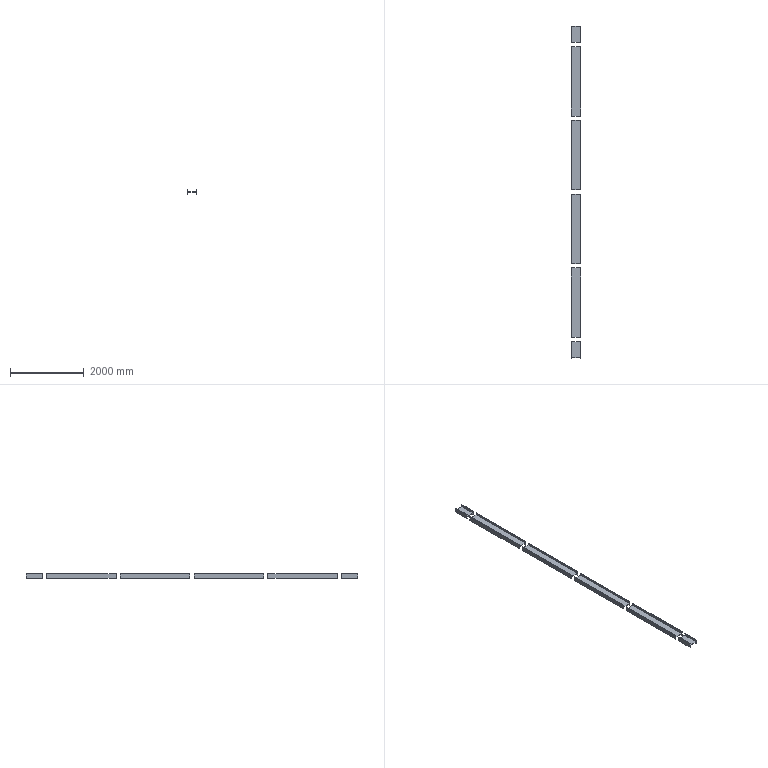Component | NX | CHUNSHUIJINCAO_DIHEN_3 | 6 solids | 84 faces | volume 44640280 mm3 | plane 84